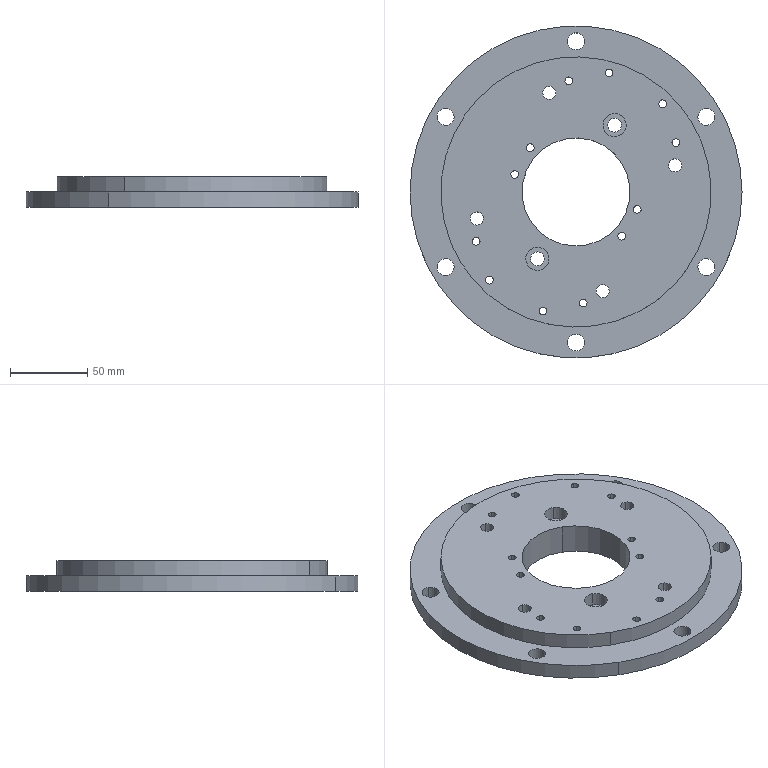Component | SolidWorks | SpindleFixtureAssemblyLeft-1_KLHFH002Turntable-2-1 | 1 solid | 69 faces | box 215 x 215 x 20 mm | volume 506250 mm3 | cylinder 62 | plane 7 | commonest cylinder face diameters 5 x24 11 x12 8.5 x8 16 x4 15 x4 9 x4 175 x2 70 x2 | material Plain Carbon Steel
build123d program:
from build123d import *

# Parameters (mm, degrees)
SKETCH1_R                                          = 265
BOSS_EXTRUDE1_DEPTH                                = 10
SKETCH2_R                                          = 30
SKETCH2_R_2                                        = 35
CUT_EXTRUDE1_DEPTH                                 = 376.3
HOLE_SIZE_ACCORDING_TO_TYPE_1_OF_HEXAG_D           = 13.5
HOLE_SIZE_ACCORDING_TO_TYPE_1_OF_HEXAG_DEPTH       = 38.75
HOLE_SIZE_ACCORDING_TO_TYPE_1_OF_HEXAG_CBORE_D     = 20
HOLE_SIZE_ACCORDING_TO_TYPE_1_OF_HEXAG_CBORE_DEPTH = 13
HOLE_SIZE_ACCORDING_TO_TYPE_1_OF_HEXAG_TIP         = 4.056
M8_TAPPED_HOLE1_D                                  = 6.8
SKETCH7_R                                          = 65
CUT_EXTRUDE2_DEPTH                                 = 3
HOLE_SIZE_ACCORDING_TO_TYPE_2_OF_HEXAG_D           = 9
HOLE_SIZE_ACCORDING_TO_TYPE_2_OF_HEXAG_CBORE_D     = 15
HOLE_SIZE_ACCORDING_TO_TYPE_2_OF_HEXAG_CBORE_DEPTH = 9
SKETCH10_R                                         = 8
CUT_EXTRUDE3_DEPTH                                 = 3
M6_TAPPED_HOLE2_D                                  = 5
SKETCH15_R                                         = 30
CUT_EXTRUDE4_DEPTH                                 = 5
F_25_5_25_5_DIAMETER_HOLE1_D                       = 25.5
CIRPATTERN1_COUNT                                  = 3
M10_TAPPED_HOLE1_D                                 = 8.5
SKETCH20_R                                         = 11
CUT_EXTRUDE5_DEPTH                                 = 376.3
SKETCH21_R                                         = 11
CUT_EXTRUDE6_DEPTH                                 = 376.3
BOSS_EXTRUDE2_START                                = -12.5
SKETCH22_R                                         = 280
SKETCH22_R_2                                       = 265
BOSS_EXTRUDE2_DEPTH                                = 12.5
M6_TAPPED_HOLE3_D                                  = 5
SKETCH25_OUTSIDE_W                                 = 720.442
SKETCH25_OUTSIDE_H                                 = 720.442
SKETCH25_OUTSIDE_R                                 = 107.5
CUT_EXTRUDE8_DEPTH                                 = 397.485
SKETCH26_OUTSIDE_W                                 = 277.942
SKETCH26_OUTSIDE_H                                 = 277.942
SKETCH26_OUTSIDE_R                                 = 87.5
CUT_EXTRUDE9_DEPTH                                 = 10
F_11_0_11_DIAMETER_HOLE1_D                         = 11
CIRPATTERN2_COUNT                                  = 6


with BuildPart() as part:
    # Sketch1 → Boss-Extrude1 (new, symmetric)
    with BuildSketch(Plane.XY):
        Circle(SKETCH1_R)
    extrude(amount=BOSS_EXTRUDE1_DEPTH, both=True)

    # Sketch2 → Cut-Extrude1 (cut, through all)
    with BuildSketch(Plane.XY.offset(10)):
        with Locations((-182, 0)):
            Circle(SKETCH2_R)
        Circle(SKETCH2_R_2)
    extrude(amount=-CUT_EXTRUDE1_DEPTH, mode=Mode.SUBTRACT)

    # Hole Size _according to_ Type 1 of Hexag
    with Locations(Plane(origin=(0, 0, -10), x_dir=(-1, 0, 0), z_dir=(0, 0, -1))):
        with Locations((141, 0), (182, 41), (223, 0), (182, -41)):
            CounterBoreHole(HOLE_SIZE_ACCORDING_TO_TYPE_1_OF_HEXAG_D / 2, HOLE_SIZE_ACCORDING_TO_TYPE_1_OF_HEXAG_CBORE_D / 2, HOLE_SIZE_ACCORDING_TO_TYPE_1_OF_HEXAG_CBORE_DEPTH, depth=HOLE_SIZE_ACCORDING_TO_TYPE_1_OF_HEXAG_DEPTH)
            with Locations((0, 0, -(HOLE_SIZE_ACCORDING_TO_TYPE_1_OF_HEXAG_DEPTH + HOLE_SIZE_ACCORDING_TO_TYPE_1_OF_HEXAG_TIP / 2))):  # 118° drill point
                Cone(0, HOLE_SIZE_ACCORDING_TO_TYPE_1_OF_HEXAG_D / 2, HOLE_SIZE_ACCORDING_TO_TYPE_1_OF_HEXAG_TIP, mode=Mode.SUBTRACT)

    # M8 Tapped Hole1 (through all)
    with Locations(Plane(origin=(0, 0, -10), x_dir=(-1, 0, 0), z_dir=(0, 0, -1))):
        with Locations((212, 30), (212, -30), (152, -30), (152, 30)):
            Hole(M8_TAPPED_HOLE1_D / 2)

    # Sketch7 → Cut-Extrude2 (cut)
    with BuildSketch(Plane.XY.offset(10)):
        with Locations((-182, 0)):
            Circle(SKETCH7_R)
    extrude(amount=-CUT_EXTRUDE2_DEPTH, mode=Mode.SUBTRACT)

    # Hole Size _according to_ Type 2 of Hexag (through all)
    with Locations(Plane(origin=(0, 0, -10), x_dir=(1, 0, 0), z_dir=(0, 0, -1))):
        with Locations((-50, 0), (50, 0)):
            CounterBoreHole(HOLE_SIZE_ACCORDING_TO_TYPE_2_OF_HEXAG_D / 2, HOLE_SIZE_ACCORDING_TO_TYPE_2_OF_HEXAG_CBORE_D / 2, HOLE_SIZE_ACCORDING_TO_TYPE_2_OF_HEXAG_CBORE_DEPTH)

    # Sketch10 → Cut-Extrude3 (cut)
    with BuildSketch(Plane.XY.offset(10)):
        with Locations((-50, 0)):
            Circle(SKETCH10_R)
        with Locations((50, 0)):
            Circle(SKETCH10_R)
    extrude(amount=-CUT_EXTRUDE3_DEPTH, mode=Mode.SUBTRACT)

    # M6 Tapped Hole2 (through all)
    with Locations(Plane.XY.offset(10)):
        with Locations((-60, -40), (-77.5, -20), (-77.5, 20), (-60, 40), (10, 40), (-10, 40), (10, -40), (-10, -40), (60, -40), (77.5, -20), (77.5, 20), (60, 40)):
            Hole(M6_TAPPED_HOLE2_D / 2)

    # Sketch15 → Cut-Extrude4 (cut)
    with BuildSketch(Plane(origin=(0, 0, -10), x_dir=(-1, 0, 0), z_dir=(0, 0, -1))):
        with Locations((-220, 0)):
            Circle(SKETCH15_R)
    cut_extrude4 = extrude(amount=-CUT_EXTRUDE4_DEPTH, mode=Mode.SUBTRACT)

    # 25.5 _25.5_ Diameter Hole1 (through all)
    with Locations(Plane.XY.offset(10)):
        with Locations((220, 0)):
            f_25_5_25_5_diameter_hole1 = Hole(F_25_5_25_5_DIAMETER_HOLE1_D / 2)

    # CirPattern1: Cut-Extrude4, 25.5 _25.5_ Diameter Hole1 ×3 about axis
    cirpattern1_axis = Axis((0, 0, 0), (0, 0, 1))
    add([cut_extrude4.rotate(cirpattern1_axis, i * 360 / CIRPATTERN1_COUNT) for i in range(1, CIRPATTERN1_COUNT)], mode=Mode.SUBTRACT)
    add([f_25_5_25_5_diameter_hole1.rotate(cirpattern1_axis, i * 360 / CIRPATTERN1_COUNT) for i in range(1, CIRPATTERN1_COUNT)], mode=Mode.SUBTRACT)

    # M10 Tapped Hole1 (through all)
    with Locations(Plane(origin=(0, 0, -10), x_dir=(-1, 0, 0), z_dir=(0, 0, -1))):
        with Locations((-47, 47), (47, 47), (-47, -47), (47, -47)):
            Hole(M10_TAPPED_HOLE1_D / 2)

    # Sketch20 → Cut-Extrude5 (cut, through all)
    with BuildSketch(Plane.XY.offset(10)):
        with Locations((130, 65)):
            Circle(SKETCH20_R)
        with Locations((130, -65)):
            Circle(SKETCH20_R)
    extrude(amount=-CUT_EXTRUDE5_DEPTH, mode=Mode.SUBTRACT)

    # Sketch21 → Cut-Extrude6 (cut, through all)
    with BuildSketch(Plane.XY.offset(10)):
        with Locations((-180, -120)):
            Circle(SKETCH21_R)
        with Locations((-180, 120)):
            Circle(SKETCH21_R)
    extrude(amount=-CUT_EXTRUDE6_DEPTH, mode=Mode.SUBTRACT)

    # Sketch22 → Boss-Extrude2 (add)
    with BuildSketch(Plane(origin=(0, 0, -10), x_dir=(-1, 0, 0), z_dir=(0, 0, -1)).offset(BOSS_EXTRUDE2_START)):
        Circle(SKETCH22_R)
        Circle(SKETCH22_R_2, mode=Mode.SUBTRACT)
    extrude(amount=BOSS_EXTRUDE2_DEPTH)

    # M6 Tapped Hole3 (through all)
    with Locations(Plane.XY.offset(2.5)):
        with Locations((0, -273), (272.834, -9.528), (272.834, 9.528), (-272.834, -9.528), (-273, 9.533), (0, 273)):
            Hole(M6_TAPPED_HOLE3_D / 2)

    # Sketch25 outside → Cut-Extrude8 (cut, through all)
    with BuildSketch(Plane.XY.offset(10)):
        Rectangle(SKETCH25_OUTSIDE_W, SKETCH25_OUTSIDE_H)
        Circle(SKETCH25_OUTSIDE_R, mode=Mode.SUBTRACT)
    extrude(amount=-CUT_EXTRUDE8_DEPTH, mode=Mode.SUBTRACT)

    # Sketch26 outside → Cut-Extrude9 (cut)
    with BuildSketch(Plane(origin=(0, 0, -10), x_dir=(-1, 0, 0), z_dir=(0, 0, -1))):
        Rectangle(SKETCH26_OUTSIDE_W, SKETCH26_OUTSIDE_H)
        Circle(SKETCH26_OUTSIDE_R, mode=Mode.SUBTRACT)
    extrude(amount=-CUT_EXTRUDE9_DEPTH, mode=Mode.SUBTRACT)

    # 11.0 _11_ Diameter Hole1 (through all)
    with Locations(Plane.XY.offset(10)):
        with Locations((0, -97.5)):
            f_11_0_11_diameter_hole1 = Hole(F_11_0_11_DIAMETER_HOLE1_D / 2)

    # CirPattern2: 11.0 _11_ Diameter Hole1 ×6 about axis
    cirpattern2_axis = Axis((0, 0, 0), (0, 0, 1))
    for i in range(1, CIRPATTERN2_COUNT):
        add(f_11_0_11_diameter_hole1.rotate(cirpattern2_axis, i * 360 / CIRPATTERN2_COUNT), mode=Mode.SUBTRACT)


solid = part.part

# Placed as in the assembly
solid = solid.moved(Location((0, 0, -177.5), (180, 0, -60)))